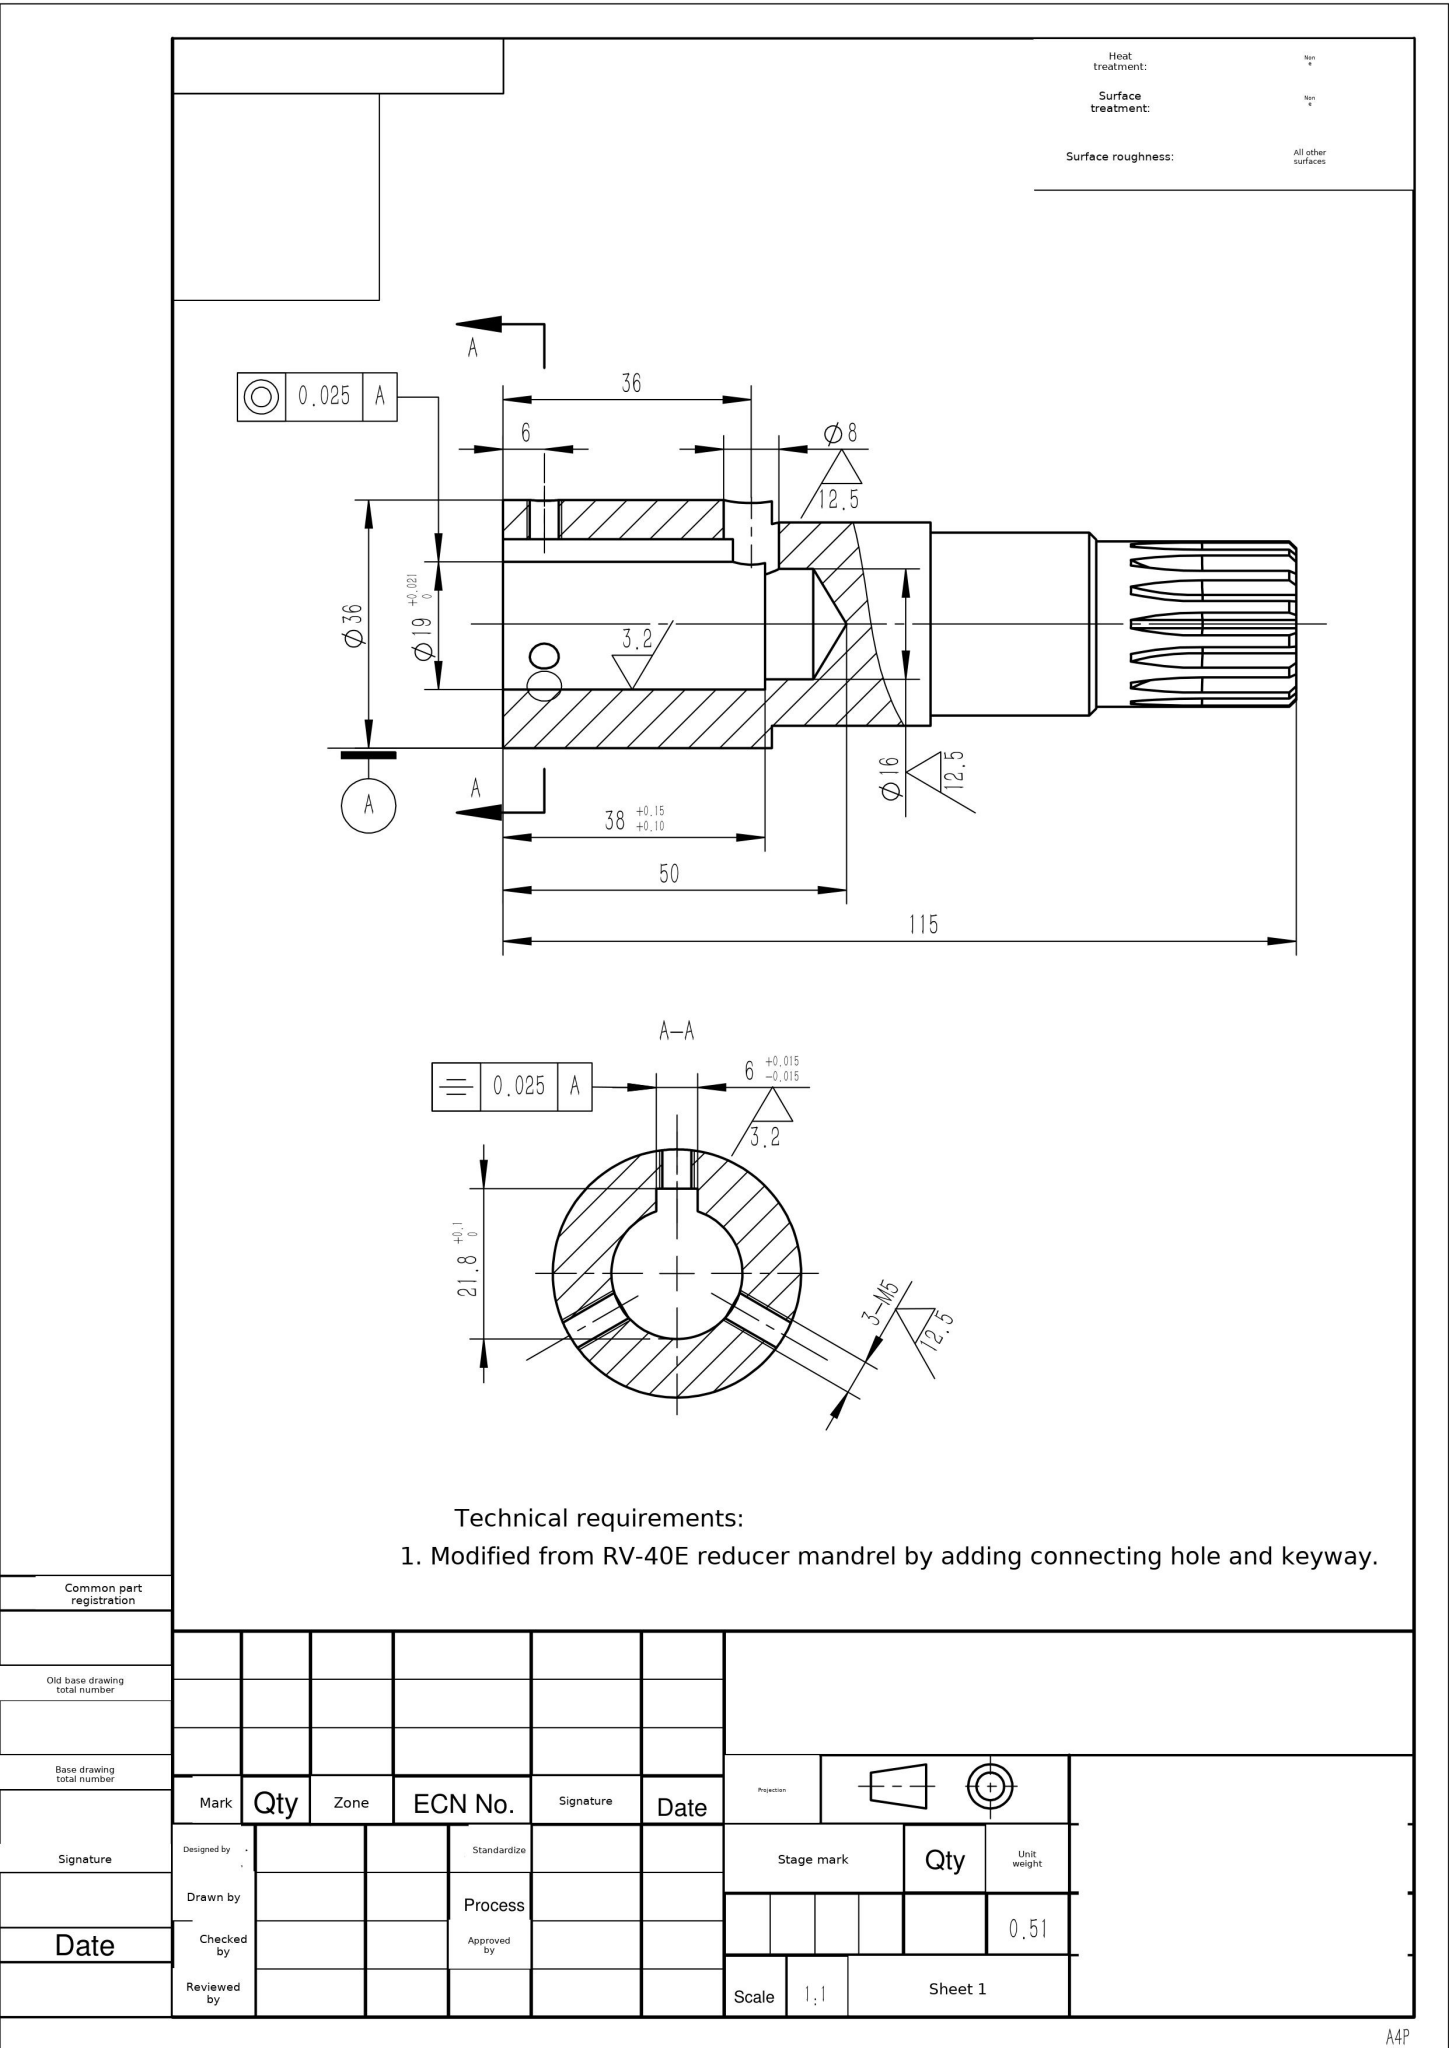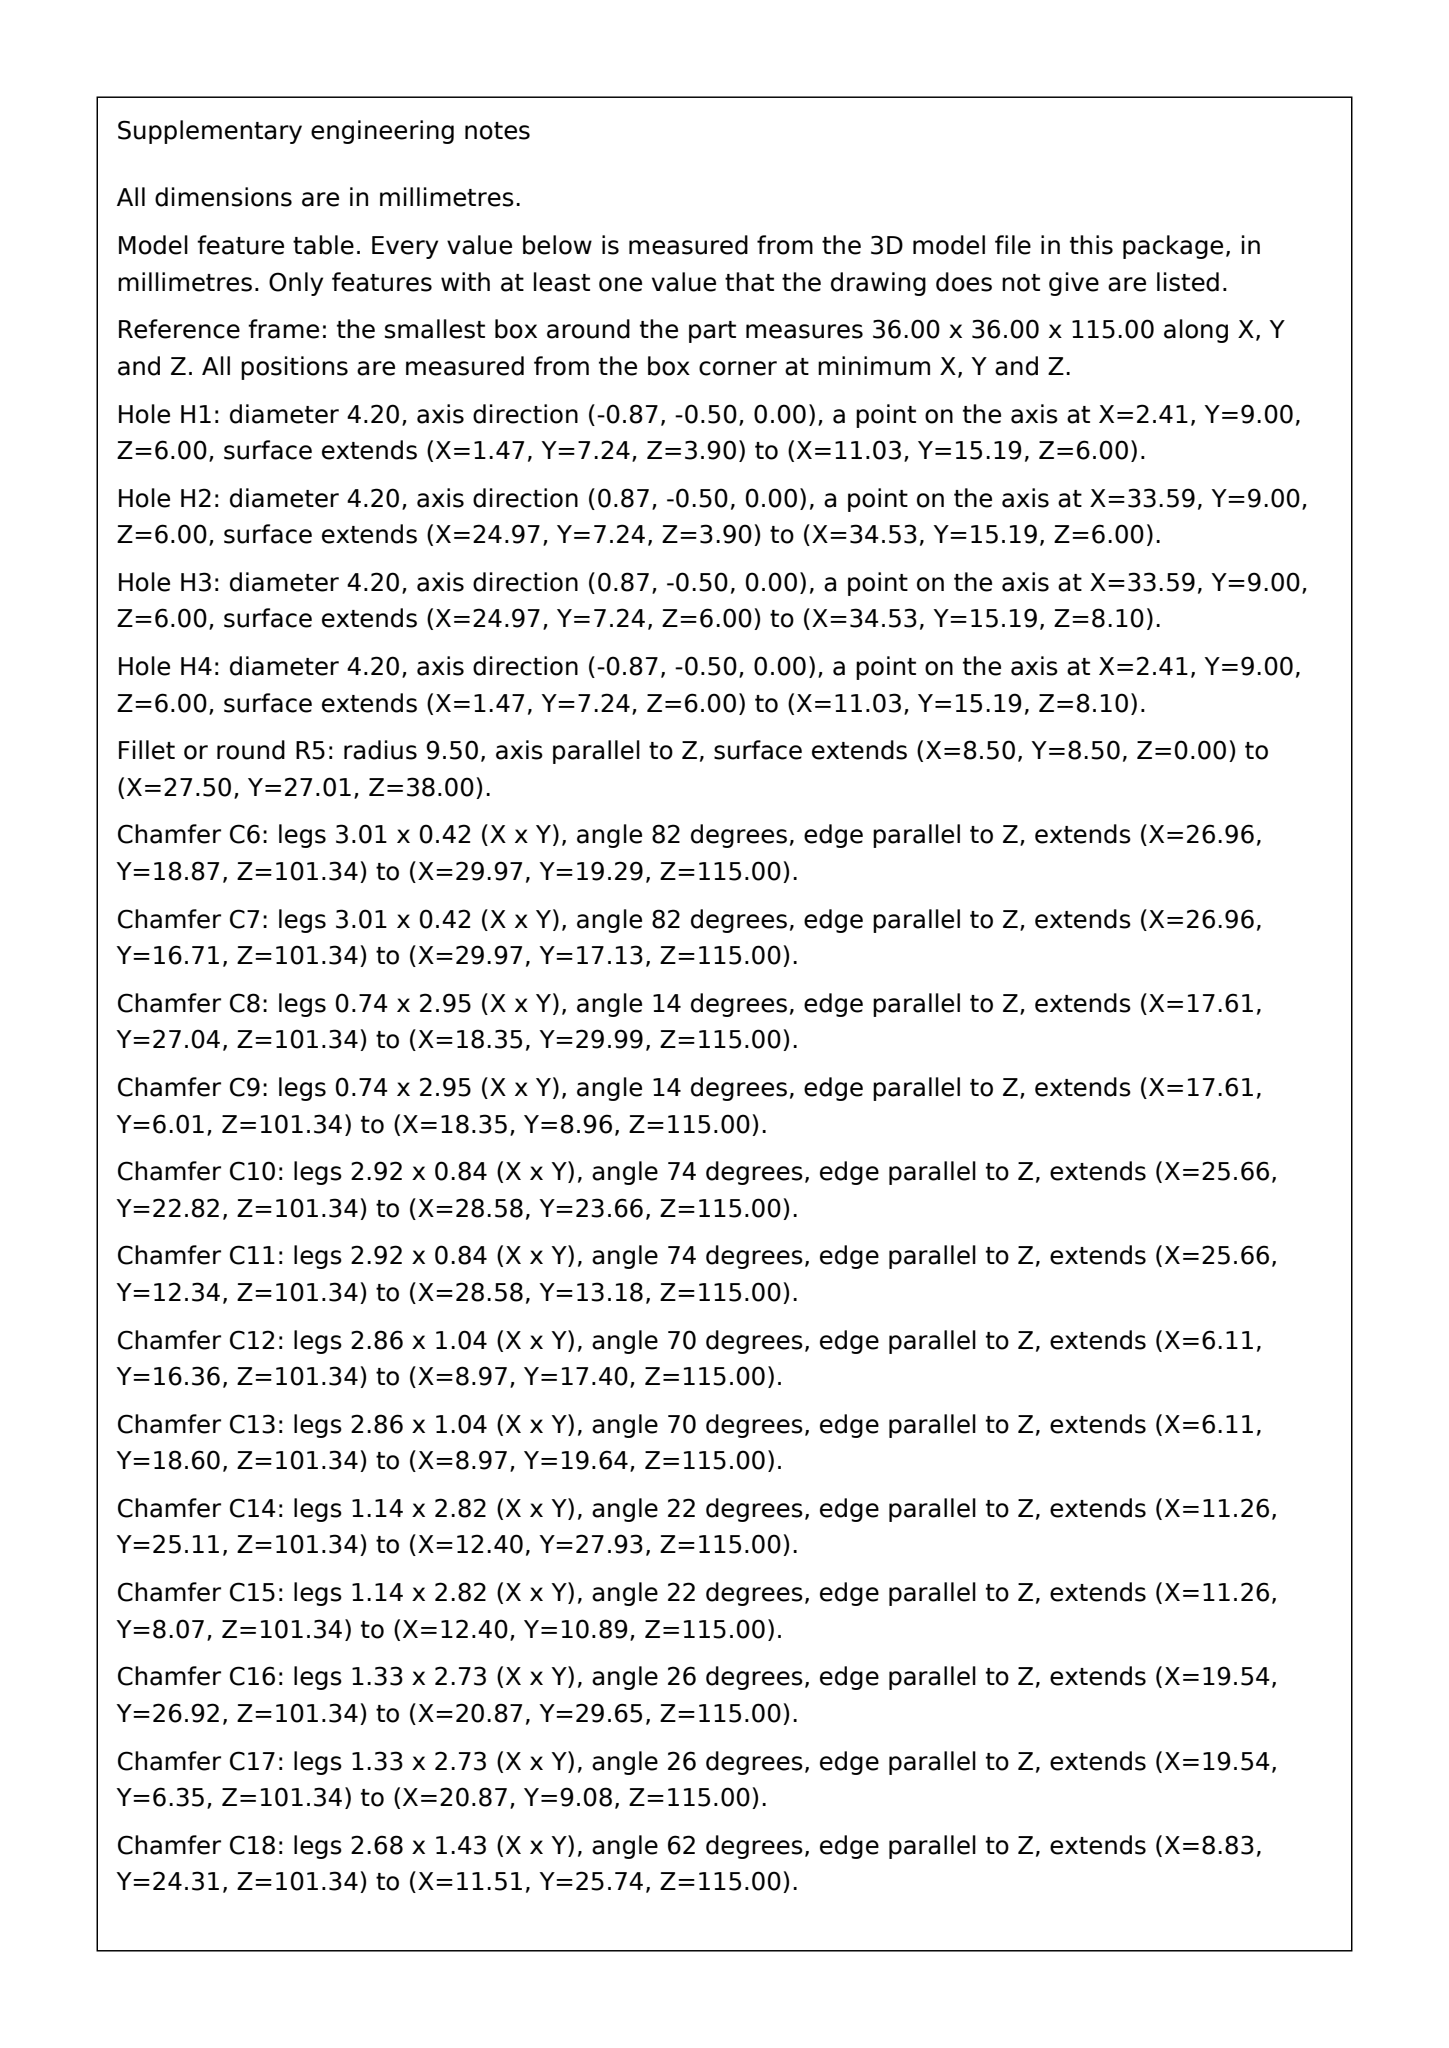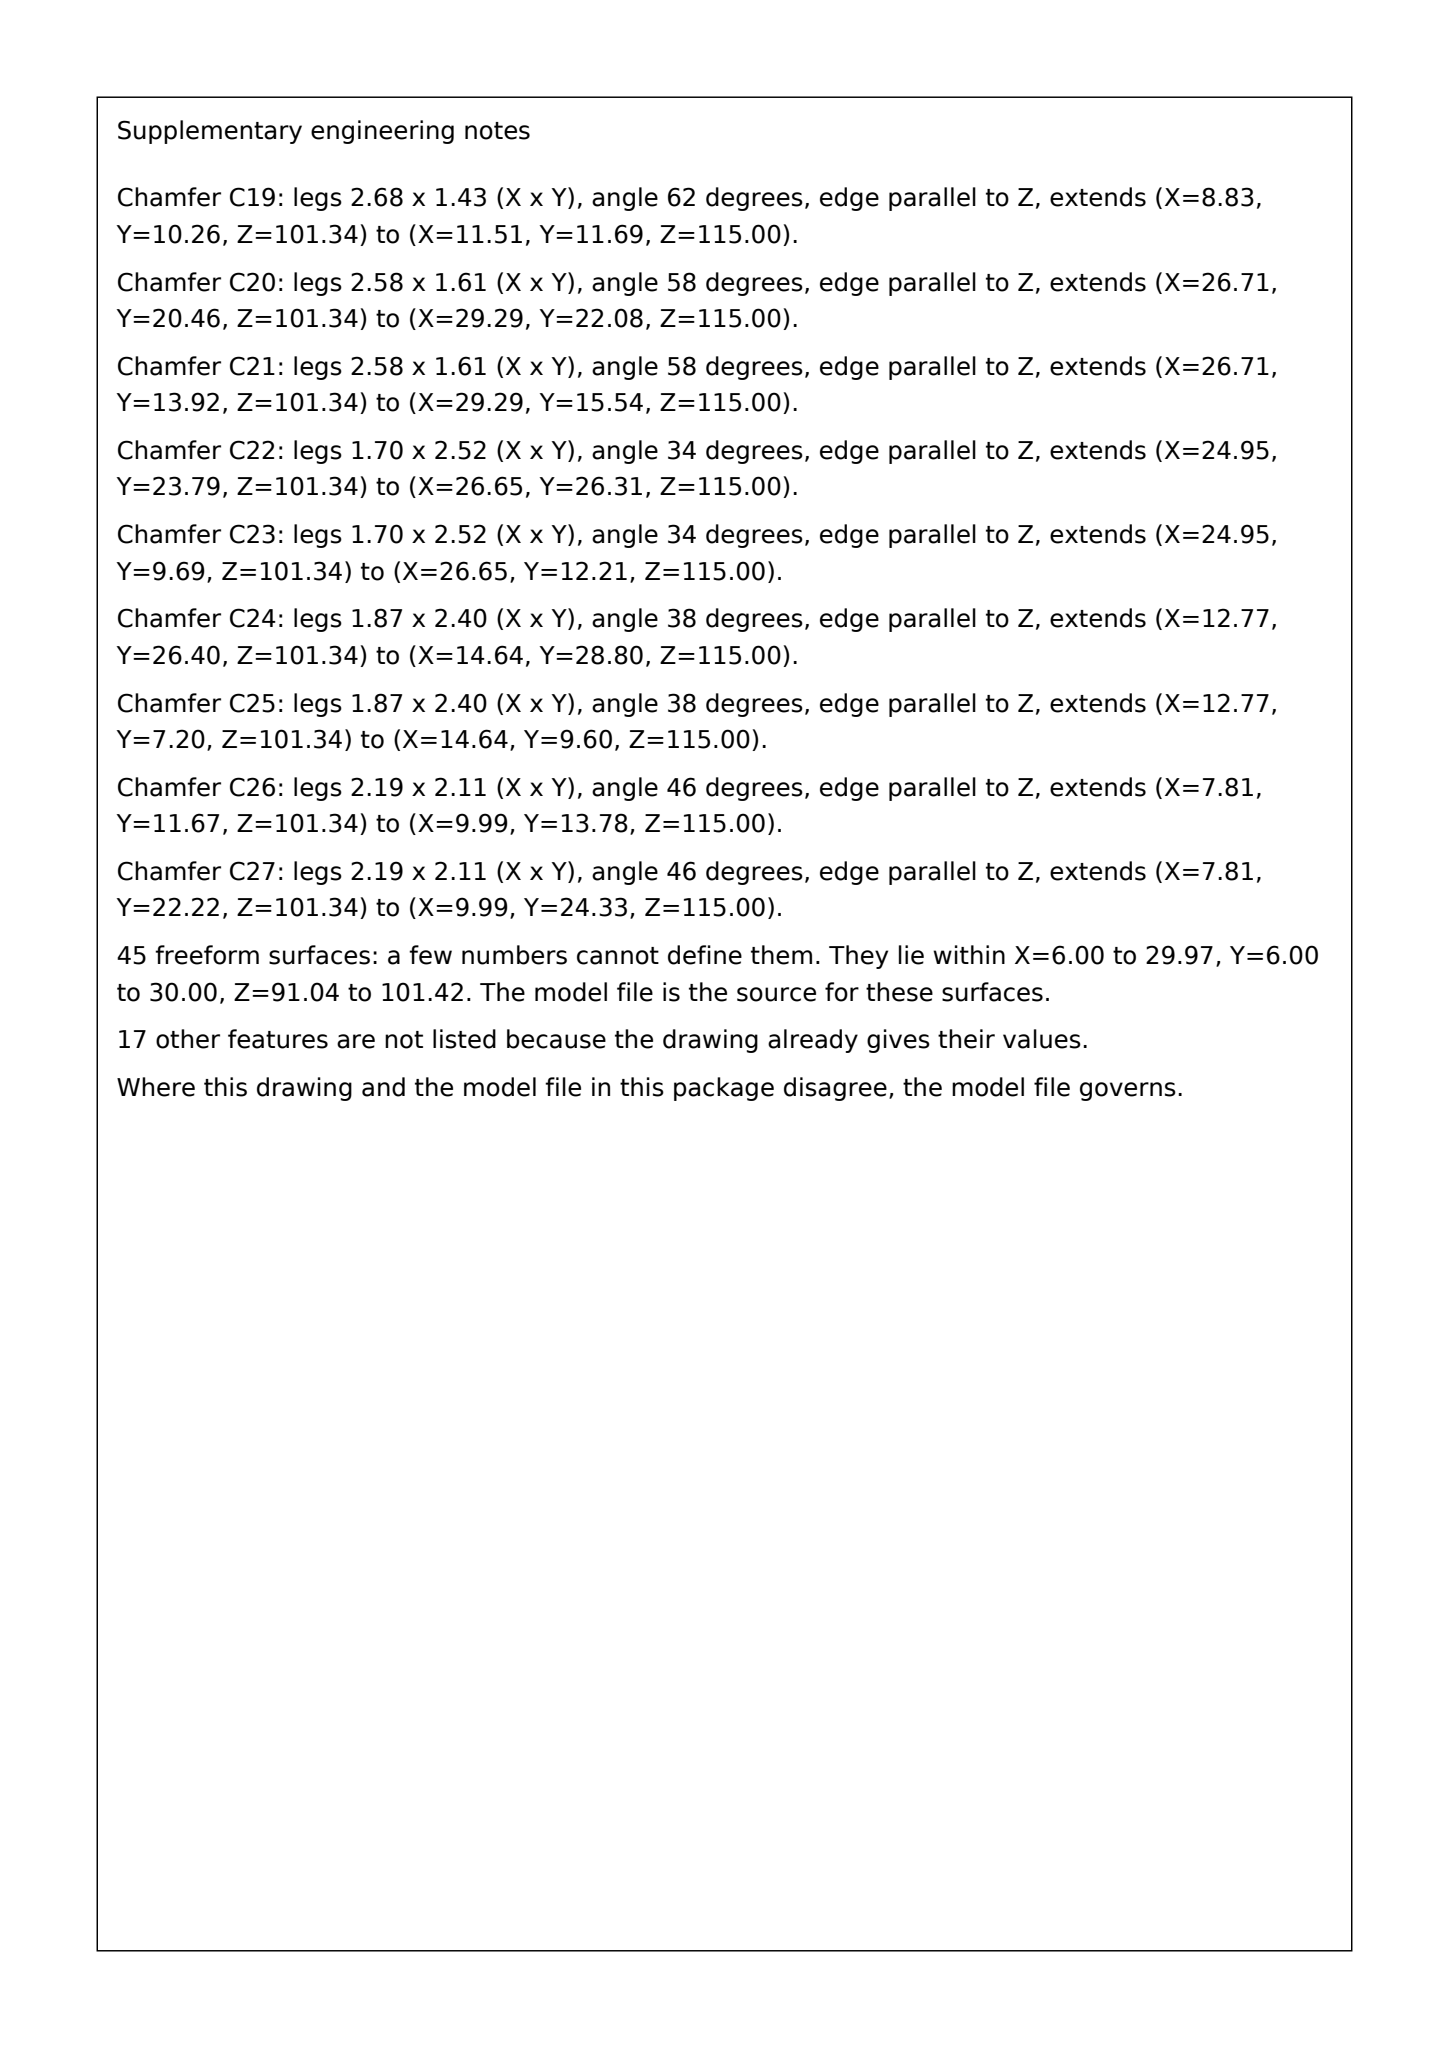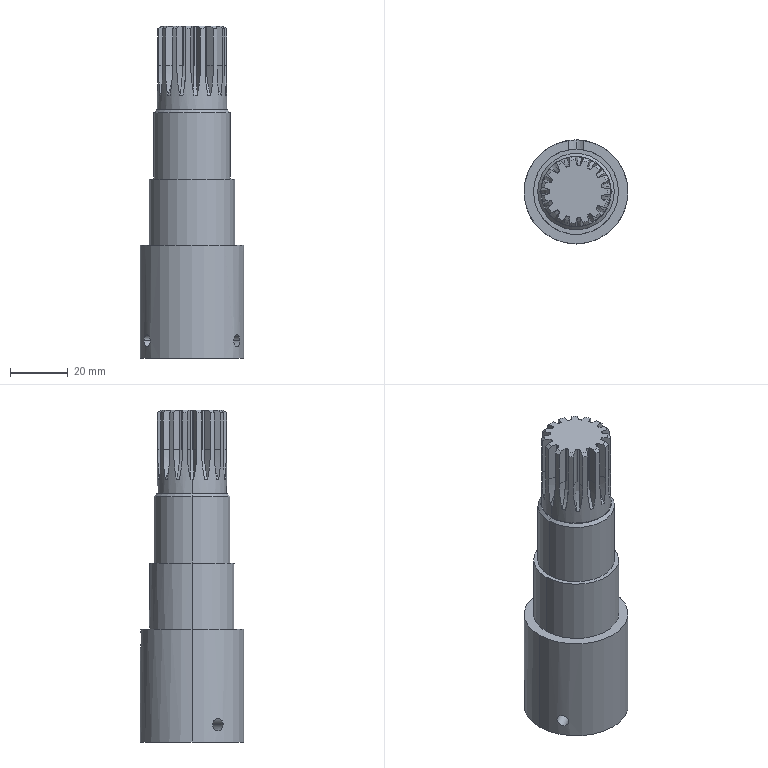Part | SolidWorks | mm | 1 solid | 154 faces | box 36 x 36 x 115 mm | volume 65861 mm3 | cylinder 51 | spline 45 | plane 39 | cone 19 | commonest cylinder face diameters 18.1 x30 4.2 x6 19 x3 8 x2 26.5 x2 24 x2 16 x2 36 x2